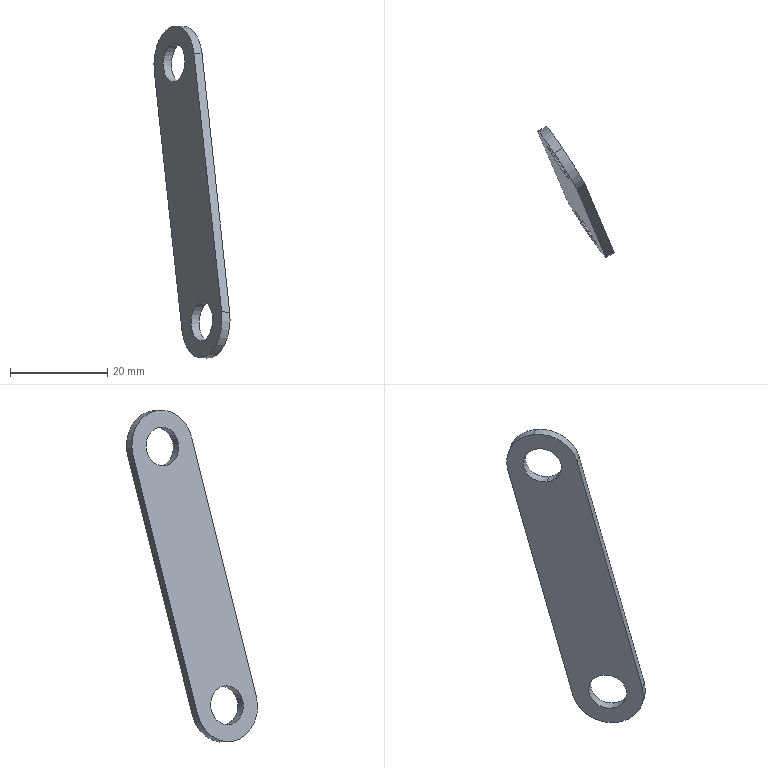Component | SolidWorks | DoorConnectionPiece-1 | 1 solid | 11 faces | box 15.63 x 26.89 x 68.15 mm | volume 1802 mm3 | cylinder 7 | plane 4 | commonest cylinder face diameters 8 x4 15 x3 | material AISI 304
build123d program:
from build123d import *

# Parameters (mm, degrees)
SKETCH1_R           = 4
BOSS_EXTRUDE1_DEPTH = 2


with BuildPart() as part:
    # Sketch1 → Boss-Extrude1 (new body)
    with BuildSketch(Plane.XY):
        with BuildLine():
            Line((0, 7.5), (55, 7.5))
            ThreePointArc((55, 7.5), (62.5, 0), (55, -7.5))
            Line((55, -7.5), (0, -7.5))
            ThreePointArc((0, -7.5), (-7.5, 0), (0, 7.5))
        make_face()
        Circle(SKETCH1_R, mode=Mode.SUBTRACT)
        with Locations((55, 0)):
            Circle(SKETCH1_R, mode=Mode.SUBTRACT)
    extrude(amount=BOSS_EXTRUDE1_DEPTH)


solid = part.part

# Placed as in the assembly
solid = solid.moved(Location((-96.017, 125.554, 686.99), (-94.979, 56.519, -100.803)))
STEP:
#1=COLOUR_RGB('',0.7922,0.8196,0.9333);
#2=FILL_AREA_STYLE_COLOUR('',#1);
#3=FILL_AREA_STYLE('',(#2));
#4=SURFACE_STYLE_FILL_AREA(#3);
#5=SURFACE_SIDE_STYLE('',(#4));
#6=SURFACE_STYLE_USAGE(.BOTH.,#5);
#7=PRESENTATION_STYLE_ASSIGNMENT((#6));
#8=CARTESIAN_POINT('',(-3.796,4.981,27.199));
#9=VERTEX_POINT('',#8);
#10=CARTESIAN_POINT('',(-3.764,4.905,26.895));
#11=VERTEX_POINT('',#10);
#12=CARTESIAN_POINT('',(-3.78,4.943,27.047));
#13=DIRECTION('',(-0.8341,-0.5496,0.04788));
#14=DIRECTION('',(0.1034,-0.241,-0.965));
#15=AXIS2_PLACEMENT_3D('',#12,#13,#14);
#16=CIRCLE('',#15,0.1575);
#17=EDGE_CURVE('',#9,#11,#16,.T.);
#18=ORIENTED_EDGE('',*,*,#17,.T.);
#19=CARTESIAN_POINT('',(-3.698,4.948,26.891));
#20=VERTEX_POINT('',#19);
#21=CARTESIAN_POINT('',(-3.764,4.905,26.895));
#22=DIRECTION('',(0.8341,0.5496,-0.04788));
#23=VECTOR('',#22,39.37);
#24=LINE('',#21,#23);
#25=EDGE_CURVE('',#11,#20,#24,.T.);
#26=ORIENTED_EDGE('',*,*,#25,.T.);
#27=CARTESIAN_POINT('',(-3.731,5.024,27.195));
#28=VERTEX_POINT('',#27);
#29=CARTESIAN_POINT('',(-3.715,4.986,27.043));
#30=DIRECTION('',(-0.8341,-0.5496,0.04788));
#31=DIRECTION('',(0.1034,-0.241,-0.965));
#32=AXIS2_PLACEMENT_3D('',#29,#30,#31);
#33=CIRCLE('',#32,0.1575);
#34=EDGE_CURVE('',#28,#20,#33,.T.);
#35=ORIENTED_EDGE('',*,*,#34,.F.);
#36=CARTESIAN_POINT('',(-3.796,4.981,27.199));
#37=DIRECTION('',(0.8341,0.5496,-0.04788));
#38=VECTOR('',#37,39.37);
#39=LINE('',#36,#38);
#40=EDGE_CURVE('',#9,#28,#39,.T.);
#41=ORIENTED_EDGE('',*,*,#40,.F.);
#42=EDGE_LOOP('',(#18,#26,#35,#41));
#43=FACE_OUTER_BOUND('',#42,.T.);
#44=CARTESIAN_POINT('',(-3.78,4.943,27.047));
#45=DIRECTION('',(0.8341,0.5496,-0.04788));
#46=DIRECTION('',(-0.1034,0.241,0.965));
#47=AXIS2_PLACEMENT_3D('',#44,#45,#46);
#48=CYLINDRICAL_SURFACE('',#47,0.1575);
#49=ADVANCED_FACE('',(#43),#48,.F.);
#50=CARTESIAN_POINT('',(-4.02,5.503,29.288));
#51=VERTEX_POINT('',#50);
#52=CARTESIAN_POINT('',(-3.988,5.427,28.984));
#53=VERTEX_POINT('',#52);
#54=CARTESIAN_POINT('',(-4.004,5.465,29.136));
#55=DIRECTION('',(-0.8341,-0.5496,0.04788));
#56=DIRECTION('',(0.1034,-0.241,-0.965));
#57=AXIS2_PLACEMENT_3D('',#54,#55,#56);
#58=CIRCLE('',#57,0.1575);
#59=EDGE_CURVE('',#51,#53,#58,.T.);
#60=ORIENTED_EDGE('',*,*,#59,.T.);
#61=CARTESIAN_POINT('',(-3.922,5.47,28.981));
#62=VERTEX_POINT('',#61);
#63=CARTESIAN_POINT('',(-3.988,5.427,28.984));
#64=DIRECTION('',(0.8341,0.5496,-0.04788));
#65=VECTOR('',#64,39.37);
#66=LINE('',#63,#65);
#67=EDGE_CURVE('',#53,#62,#66,.T.);
#68=ORIENTED_EDGE('',*,*,#67,.T.);
#69=CARTESIAN_POINT('',(-3.955,5.546,29.285));
#70=VERTEX_POINT('',#69);
#71=CARTESIAN_POINT('',(-3.938,5.508,29.133));
#72=DIRECTION('',(-0.8341,-0.5496,0.04788));
#73=DIRECTION('',(0.1034,-0.241,-0.965));
#74=AXIS2_PLACEMENT_3D('',#71,#72,#73);
#75=CIRCLE('',#74,0.1575);
#76=EDGE_CURVE('',#70,#62,#75,.T.);
#77=ORIENTED_EDGE('',*,*,#76,.F.);
#78=CARTESIAN_POINT('',(-4.02,5.503,29.288));
#79=DIRECTION('',(0.8341,0.5496,-0.04788));
#80=VECTOR('',#79,39.37);
#81=LINE('',#78,#80);
#82=EDGE_CURVE('',#51,#70,#81,.T.);
#83=ORIENTED_EDGE('',*,*,#82,.F.);
#84=EDGE_LOOP('',(#60,#68,#77,#83));
#85=FACE_OUTER_BOUND('',#84,.T.);
#86=CARTESIAN_POINT('',(-4.004,5.465,29.136));
#87=DIRECTION('',(0.8341,0.5496,-0.04788));
#88=DIRECTION('',(-0.1034,0.241,0.965));
#89=AXIS2_PLACEMENT_3D('',#86,#87,#88);
#90=CYLINDRICAL_SURFACE('',#89,0.1575);
#91=ADVANCED_FACE('',(#85),#90,.F.);
#92=CARTESIAN_POINT('',(-4.035,5.536,29.421));
#93=VERTEX_POINT('',#92);
#94=CARTESIAN_POINT('',(-4.164,5.701,29.06));
#95=VERTEX_POINT('',#94);
#96=CARTESIAN_POINT('',(-4.004,5.465,29.136));
#97=DIRECTION('',(-0.8341,-0.5496,0.04788));
#98=DIRECTION('',(0.1034,-0.241,-0.965));
#99=AXIS2_PLACEMENT_3D('',#96,#97,#98);
#100=CIRCLE('',#99,0.2953);
#101=EDGE_CURVE('',#93,#95,#100,.T.);
#102=ORIENTED_EDGE('',*,*,#101,.F.);
#103=CARTESIAN_POINT('',(-3.969,5.579,29.418));
#104=VERTEX_POINT('',#103);
#105=CARTESIAN_POINT('',(-4.035,5.536,29.421));
#106=DIRECTION('',(0.8341,0.5496,-0.04788));
#107=VECTOR('',#106,39.37);
#108=LINE('',#105,#107);
#109=EDGE_CURVE('',#93,#104,#108,.T.);
#110=ORIENTED_EDGE('',*,*,#109,.T.);
#111=CARTESIAN_POINT('',(-4.098,5.744,29.057));
#112=VERTEX_POINT('',#111);
#113=CARTESIAN_POINT('',(-3.938,5.508,29.133));
#114=DIRECTION('',(-0.8341,-0.5496,0.04788));
#115=DIRECTION('',(0.1034,-0.241,-0.965));
#116=AXIS2_PLACEMENT_3D('',#113,#114,#115);
#117=CIRCLE('',#116,0.2953);
#118=EDGE_CURVE('',#104,#112,#117,.T.);
#119=ORIENTED_EDGE('',*,*,#118,.T.);
#120=CARTESIAN_POINT('',(-4.164,5.701,29.06));
#121=DIRECTION('',(0.8341,0.5496,-0.04788));
#122=VECTOR('',#121,39.37);
#123=LINE('',#120,#122);
#124=EDGE_CURVE('',#95,#112,#123,.T.);
#125=ORIENTED_EDGE('',*,*,#124,.F.);
#126=EDGE_LOOP('',(#102,#110,#119,#125));
#127=FACE_OUTER_BOUND('',#126,.T.);
#128=CARTESIAN_POINT('',(-4.004,5.465,29.136));
#129=DIRECTION('',(0.8341,0.5496,-0.04788));
#130=DIRECTION('',(-0.1034,0.241,0.965));
#131=AXIS2_PLACEMENT_3D('',#128,#129,#130);
#132=CYLINDRICAL_SURFACE('',#131,0.2953);
#133=ADVANCED_FACE('',(#127),#132,.T.);
#134=ORIENTED_EDGE('',*,*,#59,.F.);
#135=CARTESIAN_POINT('',(-4.004,5.465,29.136));
#136=DIRECTION('',(-0.8341,-0.5496,0.04788));
#137=DIRECTION('',(0.1034,-0.241,-0.965));
#138=AXIS2_PLACEMENT_3D('',#135,#136,#137);
#139=CIRCLE('',#138,0.1575);
#140=EDGE_CURVE('',#53,#51,#139,.T.);
#141=ORIENTED_EDGE('',*,*,#140,.F.);
#142=EDGE_LOOP('',(#134,#141));
#143=FACE_BOUND('',#142,.T.);
#144=CARTESIAN_POINT('',(-3.844,5.229,29.213));
#145=VERTEX_POINT('',#144);
#146=CARTESIAN_POINT('',(-4.004,5.465,29.136));
#147=DIRECTION('',(-0.8341,-0.5496,0.04788));
#148=DIRECTION('',(0.1034,-0.241,-0.965));
#149=AXIS2_PLACEMENT_3D('',#146,#147,#148);
#150=CIRCLE('',#149,0.2953);
#151=EDGE_CURVE('',#145,#93,#150,.T.);
#152=ORIENTED_EDGE('',*,*,#151,.T.);
#153=ORIENTED_EDGE('',*,*,#101,.T.);
#154=CARTESIAN_POINT('',(-3.94,5.179,26.971));
#155=VERTEX_POINT('',#154);
#156=CARTESIAN_POINT('',(-4.164,5.701,29.06));
#157=DIRECTION('',(0.1034,-0.241,-0.965));
#158=VECTOR('',#157,39.37);
#159=LINE('',#156,#158);
#160=EDGE_CURVE('',#95,#155,#159,.T.);
#161=ORIENTED_EDGE('',*,*,#160,.T.);
#162=CARTESIAN_POINT('',(-3.62,4.707,27.123));
#163=VERTEX_POINT('',#162);
#164=CARTESIAN_POINT('',(-3.78,4.943,27.047));
#165=DIRECTION('',(-0.8341,-0.5496,0.04788));
#166=DIRECTION('',(0.1034,-0.241,-0.965));
#167=AXIS2_PLACEMENT_3D('',#164,#165,#166);
#168=CIRCLE('',#167,0.2953);
#169=EDGE_CURVE('',#155,#163,#168,.T.);
#170=ORIENTED_EDGE('',*,*,#169,.T.);
#171=CARTESIAN_POINT('',(-3.844,5.229,29.213));
#172=DIRECTION('',(-0.1034,0.241,0.965));
#173=VECTOR('',#172,39.37);
#174=LINE('',#171,#173);
#175=EDGE_CURVE('',#163,#145,#174,.T.);
#176=ORIENTED_EDGE('',*,*,#175,.T.);
#177=EDGE_LOOP('',(#152,#153,#161,#170,#176));
#178=FACE_OUTER_BOUND('',#177,.T.);
#179=ORIENTED_EDGE('',*,*,#17,.F.);
#180=CARTESIAN_POINT('',(-3.78,4.943,27.047));
#181=DIRECTION('',(-0.8341,-0.5496,0.04788));
#182=DIRECTION('',(0.1034,-0.241,-0.965));
#183=AXIS2_PLACEMENT_3D('',#180,#181,#182);
#184=CIRCLE('',#183,0.1575);
#185=EDGE_CURVE('',#11,#9,#184,.T.);
#186=ORIENTED_EDGE('',*,*,#185,.F.);
#187=EDGE_LOOP('',(#179,#186));
#188=FACE_BOUND('',#187,.T.);
#189=CARTESIAN_POINT('',(-4.004,5.465,29.136));
#190=DIRECTION('',(-0.8341,-0.5496,0.04788));
#191=DIRECTION('',(0.1034,-0.241,-0.965));
#192=AXIS2_PLACEMENT_3D('',#189,#190,#191);
#193=PLANE('',#192);
#194=ADVANCED_FACE('',(#143,#178,#188),#193,.T.);
#195=ORIENTED_EDGE('',*,*,#76,.T.);
#196=CARTESIAN_POINT('',(-3.938,5.508,29.133));
#197=DIRECTION('',(-0.8341,-0.5496,0.04788));
#198=DIRECTION('',(0.1034,-0.241,-0.965));
#199=AXIS2_PLACEMENT_3D('',#196,#197,#198);
#200=CIRCLE('',#199,0.1575);
#201=EDGE_CURVE('',#62,#70,#200,.T.);
#202=ORIENTED_EDGE('',*,*,#201,.T.);
#203=EDGE_LOOP('',(#195,#202));
#204=FACE_BOUND('',#203,.T.);
#205=CARTESIAN_POINT('',(-3.778,5.272,29.209));
#206=VERTEX_POINT('',#205);
#207=CARTESIAN_POINT('',(-3.938,5.508,29.133));
#208=DIRECTION('',(-0.8341,-0.5496,0.04788));
#209=DIRECTION('',(0.1034,-0.241,-0.965));
#210=AXIS2_PLACEMENT_3D('',#207,#208,#209);
#211=CIRCLE('',#210,0.2953);
#212=EDGE_CURVE('',#206,#104,#211,.T.);
#213=ORIENTED_EDGE('',*,*,#212,.F.);
#214=CARTESIAN_POINT('',(-3.555,4.75,27.119));
#215=VERTEX_POINT('',#214);
#216=CARTESIAN_POINT('',(-3.778,5.272,29.209));
#217=DIRECTION('',(-0.1034,0.241,0.965));
#218=VECTOR('',#217,39.37);
#219=LINE('',#216,#218);
#220=EDGE_CURVE('',#215,#206,#219,.T.);
#221=ORIENTED_EDGE('',*,*,#220,.F.);
#222=CARTESIAN_POINT('',(-3.875,5.223,26.967));
#223=VERTEX_POINT('',#222);
#224=CARTESIAN_POINT('',(-3.715,4.986,27.043));
#225=DIRECTION('',(-0.8341,-0.5496,0.04788));
#226=DIRECTION('',(0.1034,-0.241,-0.965));
#227=AXIS2_PLACEMENT_3D('',#224,#225,#226);
#228=CIRCLE('',#227,0.2953);
#229=EDGE_CURVE('',#223,#215,#228,.T.);
#230=ORIENTED_EDGE('',*,*,#229,.F.);
#231=CARTESIAN_POINT('',(-4.098,5.744,29.057));
#232=DIRECTION('',(0.1034,-0.241,-0.965));
#233=VECTOR('',#232,39.37);
#234=LINE('',#231,#233);
#235=EDGE_CURVE('',#112,#223,#234,.T.);
#236=ORIENTED_EDGE('',*,*,#235,.F.);
#237=ORIENTED_EDGE('',*,*,#118,.F.);
#238=EDGE_LOOP('',(#213,#221,#230,#236,#237));
#239=FACE_OUTER_BOUND('',#238,.T.);
#240=ORIENTED_EDGE('',*,*,#34,.T.);
#241=CARTESIAN_POINT('',(-3.715,4.986,27.043));
#242=DIRECTION('',(-0.8341,-0.5496,0.04788));
#243=DIRECTION('',(0.1034,-0.241,-0.965));
#244=AXIS2_PLACEMENT_3D('',#241,#242,#243);
#245=CIRCLE('',#244,0.1575);
#246=EDGE_CURVE('',#20,#28,#245,.T.);
#247=ORIENTED_EDGE('',*,*,#246,.T.);
#248=EDGE_LOOP('',(#240,#247));
#249=FACE_BOUND('',#248,.T.);
#250=CARTESIAN_POINT('',(-3.938,5.508,29.133));
#251=DIRECTION('',(-0.8341,-0.5496,0.04788));
#252=DIRECTION('',(0.1034,-0.241,-0.965));
#253=AXIS2_PLACEMENT_3D('',#250,#251,#252);
#254=PLANE('',#253);
#255=ADVANCED_FACE('',(#204,#239,#249),#254,.F.);
#256=ORIENTED_EDGE('',*,*,#109,.F.);
#257=ORIENTED_EDGE('',*,*,#151,.F.);
#258=CARTESIAN_POINT('',(-3.844,5.229,29.213));
#259=DIRECTION('',(0.8341,0.5496,-0.04788));
#260=VECTOR('',#259,39.37);
#261=LINE('',#258,#260);
#262=EDGE_CURVE('',#145,#206,#261,.T.);
#263=ORIENTED_EDGE('',*,*,#262,.T.);
#264=ORIENTED_EDGE('',*,*,#212,.T.);
#265=EDGE_LOOP('',(#256,#257,#263,#264));
#266=FACE_OUTER_BOUND('',#265,.T.);
#267=CARTESIAN_POINT('',(-4.004,5.465,29.136));
#268=DIRECTION('',(0.8341,0.5496,-0.04788));
#269=DIRECTION('',(-0.1034,0.241,0.965));
#270=AXIS2_PLACEMENT_3D('',#267,#268,#269);
#271=CYLINDRICAL_SURFACE('',#270,0.2953);
#272=ADVANCED_FACE('',(#266),#271,.T.);
#273=ORIENTED_EDGE('',*,*,#235,.T.);
#274=CARTESIAN_POINT('',(-3.94,5.179,26.971));
#275=DIRECTION('',(0.8341,0.5496,-0.04788));
#276=VECTOR('',#275,39.37);
#277=LINE('',#274,#276);
#278=EDGE_CURVE('',#155,#223,#277,.T.);
#279=ORIENTED_EDGE('',*,*,#278,.F.);
#280=ORIENTED_EDGE('',*,*,#160,.F.);
#281=ORIENTED_EDGE('',*,*,#124,.T.);
#282=EDGE_LOOP('',(#273,#279,#280,#281));
#283=FACE_OUTER_BOUND('',#282,.T.);
#284=CARTESIAN_POINT('',(-4.164,5.701,29.06));
#285=DIRECTION('',(0.5419,-0.7999,0.2578));
#286=DIRECTION('',(-0.8341,-0.5496,0.04788));
#287=AXIS2_PLACEMENT_3D('',#284,#285,#286);
#288=PLANE('',#287);
#289=ADVANCED_FACE('',(#283),#288,.F.);
#290=ORIENTED_EDGE('',*,*,#229,.T.);
#291=CARTESIAN_POINT('',(-3.62,4.707,27.123));
#292=DIRECTION('',(0.8341,0.5496,-0.04788));
#293=VECTOR('',#292,39.37);
#294=LINE('',#291,#293);
#295=EDGE_CURVE('',#163,#215,#294,.T.);
#296=ORIENTED_EDGE('',*,*,#295,.F.);
#297=ORIENTED_EDGE('',*,*,#169,.F.);
#298=ORIENTED_EDGE('',*,*,#278,.T.);
#299=EDGE_LOOP('',(#290,#296,#297,#298));
#300=FACE_OUTER_BOUND('',#299,.T.);
#301=CARTESIAN_POINT('',(-3.78,4.943,27.047));
#302=DIRECTION('',(0.8341,0.5496,-0.04788));
#303=DIRECTION('',(-0.1034,0.241,0.965));
#304=AXIS2_PLACEMENT_3D('',#301,#302,#303);
#305=CYLINDRICAL_SURFACE('',#304,0.2953);
#306=ADVANCED_FACE('',(#300),#305,.T.);
#307=ORIENTED_EDGE('',*,*,#220,.T.);
#308=ORIENTED_EDGE('',*,*,#262,.F.);
#309=ORIENTED_EDGE('',*,*,#175,.F.);
#310=ORIENTED_EDGE('',*,*,#295,.T.);
#311=EDGE_LOOP('',(#307,#308,#309,#310));
#312=FACE_OUTER_BOUND('',#311,.T.);
#313=CARTESIAN_POINT('',(-3.844,5.229,29.213));
#314=DIRECTION('',(-0.5419,0.7999,-0.2578));
#315=DIRECTION('',(0.8341,0.5496,-0.04788));
#316=AXIS2_PLACEMENT_3D('',#313,#314,#315);
#317=PLANE('',#316);
#318=ADVANCED_FACE('',(#312),#317,.F.);
#319=ORIENTED_EDGE('',*,*,#67,.F.);
#320=ORIENTED_EDGE('',*,*,#140,.T.);
#321=ORIENTED_EDGE('',*,*,#82,.T.);
#322=ORIENTED_EDGE('',*,*,#201,.F.);
#323=EDGE_LOOP('',(#319,#320,#321,#322));
#324=FACE_OUTER_BOUND('',#323,.T.);
#325=CARTESIAN_POINT('',(-4.004,5.465,29.136));
#326=DIRECTION('',(0.8341,0.5496,-0.04788));
#327=DIRECTION('',(-0.1034,0.241,0.965));
#328=AXIS2_PLACEMENT_3D('',#325,#326,#327);
#329=CYLINDRICAL_SURFACE('',#328,0.1575);
#330=ADVANCED_FACE('',(#324),#329,.F.);
#331=ORIENTED_EDGE('',*,*,#25,.F.);
#332=ORIENTED_EDGE('',*,*,#185,.T.);
#333=ORIENTED_EDGE('',*,*,#40,.T.);
#334=ORIENTED_EDGE('',*,*,#246,.F.);
#335=EDGE_LOOP('',(#331,#332,#333,#334));
#336=FACE_OUTER_BOUND('',#335,.T.);
#337=CARTESIAN_POINT('',(-3.78,4.943,27.047));
#338=DIRECTION('',(0.8341,0.5496,-0.04788));
#339=DIRECTION('',(-0.1034,0.241,0.965));
#340=AXIS2_PLACEMENT_3D('',#337,#338,#339);
#341=CYLINDRICAL_SURFACE('',#340,0.1575);
#342=ADVANCED_FACE('',(#336),#341,.F.);
#343=CLOSED_SHELL('',(#49,#91,#133,#194,#255,#272,#289,#306,#318,#330,#342));
#344=MANIFOLD_SOLID_BREP('',#343);
#345=STYLED_ITEM('',(#7),#344);
#346=(LENGTH_UNIT()NAMED_UNIT(*)SI_UNIT($,.METRE.));
#347=LENGTH_MEASURE_WITH_UNIT(LENGTH_MEASURE(0.0254),#346);
#348=DIMENSIONAL_EXPONENTS(1.,0.,0.,0.,0.,0.,0.);
#349=(CONVERSION_BASED_UNIT('',#347)LENGTH_UNIT()NAMED_UNIT(#348));
#350=UNCERTAINTY_MEASURE_WITH_UNIT(LENGTH_MEASURE(0.00001),#349,'','');
#351=(NAMED_UNIT(*)PLANE_ANGLE_UNIT()SI_UNIT($,.RADIAN.));
#352=(NAMED_UNIT(*)SI_UNIT($,.STERADIAN.)SOLID_ANGLE_UNIT());
#353=(GEOMETRIC_REPRESENTATION_CONTEXT(3)GLOBAL_UNCERTAINTY_ASSIGNED_CONTEXT((#350))GLOBAL_UNIT_ASSIGNED_CONTEXT((#349,#351,#352))REPRESENTATION_CONTEXT('',''));
#354=MECHANICAL_DESIGN_GEOMETRIC_PRESENTATION_REPRESENTATION('',(#345),#353);
#355=PRESENTATION_LAYER_ASSIGNMENT('','',(#345));
#356=CARTESIAN_POINT('',(0.,0.,0.));
#357=DIRECTION('',(0.,0.,1.));
#358=DIRECTION('',(1.,0.,0.));
#359=AXIS2_PLACEMENT_3D('',#356,#357,#358);
#360=(LENGTH_UNIT()NAMED_UNIT(*)SI_UNIT($,.METRE.));
#361=LENGTH_MEASURE_WITH_UNIT(LENGTH_MEASURE(0.0254),#360);
#362=DIMENSIONAL_EXPONENTS(1.,0.,0.,0.,0.,0.,0.);
#363=(CONVERSION_BASED_UNIT('',#361)LENGTH_UNIT()NAMED_UNIT(#362));
#364=UNCERTAINTY_MEASURE_WITH_UNIT(LENGTH_MEASURE(0.00001),#363,'','');
#365=(NAMED_UNIT(*)PLANE_ANGLE_UNIT()SI_UNIT($,.RADIAN.));
#366=(NAMED_UNIT(*)SI_UNIT($,.STERADIAN.)SOLID_ANGLE_UNIT());
#367=(GEOMETRIC_REPRESENTATION_CONTEXT(3)GLOBAL_UNCERTAINTY_ASSIGNED_CONTEXT((#364))GLOBAL_UNIT_ASSIGNED_CONTEXT((#363,#365,#366))REPRESENTATION_CONTEXT('',''));
#368=ADVANCED_BREP_SHAPE_REPRESENTATION('',(#344,#359),#367);